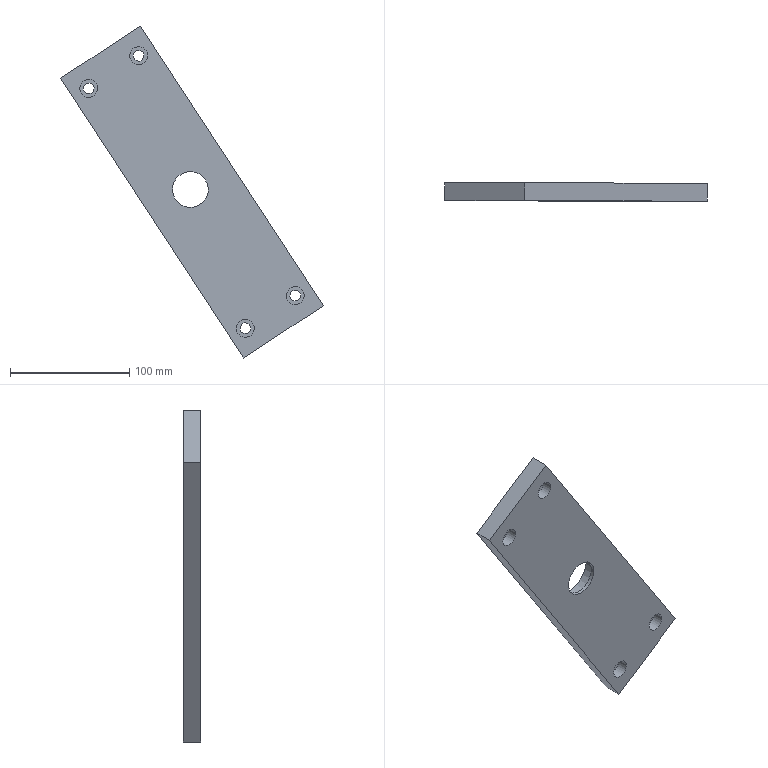Component | SolidWorks | SuctionCupRotatingShaftFixingPlate-1 | 1 solid | 31 faces | box 220.12 x 15 x 278.16 mm | volume 309366 mm3 | cylinder 20 | plane 11 | commonest cylinder face diameters 15 x8 9 x8 42 x2 30 x2 | material 6061 Alloy
build123d program:
from build123d import *

# Parameters (mm, degrees)
SKETCH1_W                                            = 80
SKETCH1_H                                            = 280
BOSS_EXTRUDE1_DEPTH                                  = 15
SKETCH2_R                                            = 15
CUT_EXTRUDE1_DEPTH                                   = 147.373
HOLE_SIZE_ACCORDING_TO_THE_TYPE_OF_HEXAG_D           = 9
HOLE_SIZE_ACCORDING_TO_THE_TYPE_OF_HEXAG_CBORE_D     = 15
HOLE_SIZE_ACCORDING_TO_THE_TYPE_OF_HEXAG_CBORE_DEPTH = 9
SKETCH5_R                                            = 21
CUT_EXTRUDE2_DEPTH                                   = 12


with BuildPart() as part:
    # Sketch1 → Boss-Extrude1 (new body)
    with BuildSketch(Plane.XY):
        Rectangle(SKETCH1_W, SKETCH1_H)
    extrude(amount=BOSS_EXTRUDE1_DEPTH)

    # Sketch2 → Cut-Extrude1 (cut, through all)
    with BuildSketch(Plane.XY.offset(15)):
        with Locations((0, 2.5)):
            Circle(SKETCH2_R)
    extrude(amount=-CUT_EXTRUDE1_DEPTH, mode=Mode.SUBTRACT)

    # Hole Size according to the type of hexag (through all)
    with Locations(Plane.XY.offset(15)):
        with Locations((-25, 120), (25, 120), (25, -120), (-25, -120)):
            CounterBoreHole(HOLE_SIZE_ACCORDING_TO_THE_TYPE_OF_HEXAG_D / 2, HOLE_SIZE_ACCORDING_TO_THE_TYPE_OF_HEXAG_CBORE_D / 2, HOLE_SIZE_ACCORDING_TO_THE_TYPE_OF_HEXAG_CBORE_DEPTH)

    # Sketch5 → Cut-Extrude2 (cut)
    with BuildSketch(Plane(origin=(0, 0, 0), x_dir=(-1, 0, 0), z_dir=(0, 0, -1))):
        with Locations((0, 2.5)):
            Circle(SKETCH5_R)
    extrude(amount=-CUT_EXTRUDE2_DEPTH, mode=Mode.SUBTRACT)


solid = part.part

# Placed as in the assembly
solid = solid.moved(Location((-27.318, 319.546, 8.337), (90, 0, 33.158)))
STEP:
#1=CARTESIAN_POINT('',(-0.4372,12.108,0.8628));
#2=VERTEX_POINT('',#1);
#3=CARTESIAN_POINT('',(-1.821,12.108,-0.04158));
#4=VERTEX_POINT('',#3);
#5=CARTESIAN_POINT('',(-1.129,12.108,0.4106));
#6=DIRECTION('',(0.,1.,-0.));
#7=DIRECTION('',(-0.8372,0.,-0.5469));
#8=AXIS2_PLACEMENT_3D('',#5,#6,#7);
#9=CIRCLE('',#8,0.8268);
#10=EDGE_CURVE('',#2,#4,#9,.T.);
#11=ORIENTED_EDGE('',*,*,#10,.F.);
#12=CARTESIAN_POINT('',(-0.4372,12.581,0.8628));
#13=VERTEX_POINT('',#12);
#14=CARTESIAN_POINT('',(-0.4372,12.108,0.8628));
#15=DIRECTION('',(0.,1.,-0.));
#16=VECTOR('',#15,39.37);
#17=LINE('',#14,#16);
#18=EDGE_CURVE('',#2,#13,#17,.T.);
#19=ORIENTED_EDGE('',*,*,#18,.T.);
#20=CARTESIAN_POINT('',(-1.821,12.581,-0.04158));
#21=VERTEX_POINT('',#20);
#22=CARTESIAN_POINT('',(-1.129,12.581,0.4106));
#23=DIRECTION('',(0.,1.,-0.));
#24=DIRECTION('',(-0.8372,0.,-0.5469));
#25=AXIS2_PLACEMENT_3D('',#22,#23,#24);
#26=CIRCLE('',#25,0.8268);
#27=EDGE_CURVE('',#13,#21,#26,.T.);
#28=ORIENTED_EDGE('',*,*,#27,.T.);
#29=CARTESIAN_POINT('',(-1.821,12.108,-0.04158));
#30=DIRECTION('',(0.,1.,-0.));
#31=VECTOR('',#30,39.37);
#32=LINE('',#29,#31);
#33=EDGE_CURVE('',#4,#21,#32,.T.);
#34=ORIENTED_EDGE('',*,*,#33,.F.);
#35=EDGE_LOOP('',(#11,#19,#28,#34));
#36=FACE_OUTER_BOUND('',#35,.T.);
#37=CARTESIAN_POINT('',(-1.129,12.108,0.4106));
#38=DIRECTION('',(0.,1.,-0.));
#39=DIRECTION('',(-0.8372,0.,-0.5469));
#40=AXIS2_PLACEMENT_3D('',#37,#38,#39);
#41=CYLINDRICAL_SURFACE('',#40,0.8268);
#42=ADVANCED_FACE('',(#36),#41,.F.);
#43=CARTESIAN_POINT('',(-4.731,12.344,3.584));
#44=VERTEX_POINT('',#43);
#45=CARTESIAN_POINT('',(-4.236,12.344,3.907));
#46=VERTEX_POINT('',#45);
#47=CARTESIAN_POINT('',(-4.483,12.344,3.745));
#48=DIRECTION('',(-0.,-1.,0.));
#49=DIRECTION('',(0.8372,0.,0.5469));
#50=AXIS2_PLACEMENT_3D('',#47,#48,#49);
#51=CIRCLE('',#50,0.2953);
#52=EDGE_CURVE('',#44,#46,#51,.T.);
#53=ORIENTED_EDGE('',*,*,#52,.F.);
#54=CARTESIAN_POINT('',(-4.731,11.99,3.584));
#55=VERTEX_POINT('',#54);
#56=CARTESIAN_POINT('',(-4.731,11.99,3.584));
#57=DIRECTION('',(-0.,-1.,0.));
#58=VECTOR('',#57,39.37);
#59=LINE('',#56,#58);
#60=EDGE_CURVE('',#44,#55,#59,.T.);
#61=ORIENTED_EDGE('',*,*,#60,.T.);
#62=CARTESIAN_POINT('',(-4.236,11.99,3.907));
#63=VERTEX_POINT('',#62);
#64=CARTESIAN_POINT('',(-4.483,11.99,3.745));
#65=DIRECTION('',(-0.,-1.,0.));
#66=DIRECTION('',(0.8372,0.,0.5469));
#67=AXIS2_PLACEMENT_3D('',#64,#65,#66);
#68=CIRCLE('',#67,0.2953);
#69=EDGE_CURVE('',#55,#63,#68,.T.);
#70=ORIENTED_EDGE('',*,*,#69,.T.);
#71=CARTESIAN_POINT('',(-4.236,11.99,3.907));
#72=DIRECTION('',(-0.,-1.,0.));
#73=VECTOR('',#72,39.37);
#74=LINE('',#71,#73);
#75=EDGE_CURVE('',#46,#63,#74,.T.);
#76=ORIENTED_EDGE('',*,*,#75,.F.);
#77=EDGE_LOOP('',(#53,#61,#70,#76));
#78=FACE_OUTER_BOUND('',#77,.T.);
#79=CARTESIAN_POINT('',(-4.483,11.99,3.745));
#80=DIRECTION('',(-0.,-1.,0.));
#81=DIRECTION('',(0.8372,0.,0.5469));
#82=AXIS2_PLACEMENT_3D('',#79,#80,#81);
#83=CYLINDRICAL_SURFACE('',#82,0.2953);
#84=ADVANCED_FACE('',(#78),#83,.F.);
#85=CARTESIAN_POINT('',(-4.632,12.581,3.648));
#86=VERTEX_POINT('',#85);
#87=CARTESIAN_POINT('',(-4.335,12.581,3.842));
#88=VERTEX_POINT('',#87);
#89=CARTESIAN_POINT('',(-4.483,12.581,3.745));
#90=DIRECTION('',(-0.,-1.,0.));
#91=DIRECTION('',(0.8372,0.,0.5469));
#92=AXIS2_PLACEMENT_3D('',#89,#90,#91);
#93=CIRCLE('',#92,0.1772);
#94=EDGE_CURVE('',#86,#88,#93,.T.);
#95=ORIENTED_EDGE('',*,*,#94,.F.);
#96=CARTESIAN_POINT('',(-4.632,12.344,3.648));
#97=VERTEX_POINT('',#96);
#98=CARTESIAN_POINT('',(-4.632,11.99,3.648));
#99=DIRECTION('',(-0.,-1.,0.));
#100=VECTOR('',#99,39.37);
#101=LINE('',#98,#100);
#102=EDGE_CURVE('',#86,#97,#101,.T.);
#103=ORIENTED_EDGE('',*,*,#102,.T.);
#104=CARTESIAN_POINT('',(-4.335,12.344,3.842));
#105=VERTEX_POINT('',#104);
#106=CARTESIAN_POINT('',(-4.483,12.344,3.745));
#107=DIRECTION('',(-0.,-1.,0.));
#108=DIRECTION('',(0.8372,0.,0.5469));
#109=AXIS2_PLACEMENT_3D('',#106,#107,#108);
#110=CIRCLE('',#109,0.1772);
#111=EDGE_CURVE('',#97,#105,#110,.T.);
#112=ORIENTED_EDGE('',*,*,#111,.T.);
#113=CARTESIAN_POINT('',(-4.335,11.99,3.842));
#114=DIRECTION('',(-0.,-1.,0.));
#115=VECTOR('',#114,39.37);
#116=LINE('',#113,#115);
#117=EDGE_CURVE('',#88,#105,#116,.T.);
#118=ORIENTED_EDGE('',*,*,#117,.F.);
#119=EDGE_LOOP('',(#95,#103,#112,#118));
#120=FACE_OUTER_BOUND('',#119,.T.);
#121=CARTESIAN_POINT('',(-4.483,11.99,3.745));
#122=DIRECTION('',(-0.,-1.,0.));
#123=DIRECTION('',(0.8372,0.,0.5469));
#124=AXIS2_PLACEMENT_3D('',#121,#122,#123);
#125=CYLINDRICAL_SURFACE('',#124,0.1772);
#126=ADVANCED_FACE('',(#120),#125,.F.);
#127=CARTESIAN_POINT('',(-3.083,12.344,4.66));
#128=VERTEX_POINT('',#127);
#129=CARTESIAN_POINT('',(-2.588,12.344,4.983));
#130=VERTEX_POINT('',#129);
#131=CARTESIAN_POINT('',(-2.835,12.344,4.822));
#132=DIRECTION('',(-0.,-1.,0.));
#133=DIRECTION('',(0.8372,0.,0.5469));
#134=AXIS2_PLACEMENT_3D('',#131,#132,#133);
#135=CIRCLE('',#134,0.2953);
#136=EDGE_CURVE('',#128,#130,#135,.T.);
#137=ORIENTED_EDGE('',*,*,#136,.F.);
#138=CARTESIAN_POINT('',(-3.083,11.99,4.66));
#139=VERTEX_POINT('',#138);
#140=CARTESIAN_POINT('',(-3.083,11.99,4.66));
#141=DIRECTION('',(-0.,-1.,0.));
#142=VECTOR('',#141,39.37);
#143=LINE('',#140,#142);
#144=EDGE_CURVE('',#128,#139,#143,.T.);
#145=ORIENTED_EDGE('',*,*,#144,.T.);
#146=CARTESIAN_POINT('',(-2.588,11.99,4.983));
#147=VERTEX_POINT('',#146);
#148=CARTESIAN_POINT('',(-2.835,11.99,4.822));
#149=DIRECTION('',(-0.,-1.,0.));
#150=DIRECTION('',(0.8372,0.,0.5469));
#151=AXIS2_PLACEMENT_3D('',#148,#149,#150);
#152=CIRCLE('',#151,0.2953);
#153=EDGE_CURVE('',#139,#147,#152,.T.);
#154=ORIENTED_EDGE('',*,*,#153,.T.);
#155=CARTESIAN_POINT('',(-2.588,11.99,4.983));
#156=DIRECTION('',(-0.,-1.,0.));
#157=VECTOR('',#156,39.37);
#158=LINE('',#155,#157);
#159=EDGE_CURVE('',#130,#147,#158,.T.);
#160=ORIENTED_EDGE('',*,*,#159,.F.);
#161=EDGE_LOOP('',(#137,#145,#154,#160));
#162=FACE_OUTER_BOUND('',#161,.T.);
#163=CARTESIAN_POINT('',(-2.835,11.99,4.822));
#164=DIRECTION('',(-0.,-1.,0.));
#165=DIRECTION('',(0.8372,0.,0.5469));
#166=AXIS2_PLACEMENT_3D('',#163,#164,#165);
#167=CYLINDRICAL_SURFACE('',#166,0.2953);
#168=ADVANCED_FACE('',(#162),#167,.F.);
#169=CARTESIAN_POINT('',(-2.984,12.581,4.725));
#170=VERTEX_POINT('',#169);
#171=CARTESIAN_POINT('',(-2.687,12.581,4.919));
#172=VERTEX_POINT('',#171);
#173=CARTESIAN_POINT('',(-2.835,12.581,4.822));
#174=DIRECTION('',(-0.,-1.,0.));
#175=DIRECTION('',(0.8372,0.,0.5469));
#176=AXIS2_PLACEMENT_3D('',#173,#174,#175);
#177=CIRCLE('',#176,0.1772);
#178=EDGE_CURVE('',#170,#172,#177,.T.);
#179=ORIENTED_EDGE('',*,*,#178,.F.);
#180=CARTESIAN_POINT('',(-2.984,12.344,4.725));
#181=VERTEX_POINT('',#180);
#182=CARTESIAN_POINT('',(-2.984,11.99,4.725));
#183=DIRECTION('',(-0.,-1.,0.));
#184=VECTOR('',#183,39.37);
#185=LINE('',#182,#184);
#186=EDGE_CURVE('',#170,#181,#185,.T.);
#187=ORIENTED_EDGE('',*,*,#186,.T.);
#188=CARTESIAN_POINT('',(-2.687,12.344,4.919));
#189=VERTEX_POINT('',#188);
#190=CARTESIAN_POINT('',(-2.835,12.344,4.822));
#191=DIRECTION('',(-0.,-1.,0.));
#192=DIRECTION('',(0.8372,0.,0.5469));
#193=AXIS2_PLACEMENT_3D('',#190,#191,#192);
#194=CIRCLE('',#193,0.1772);
#195=EDGE_CURVE('',#181,#189,#194,.T.);
#196=ORIENTED_EDGE('',*,*,#195,.T.);
#197=CARTESIAN_POINT('',(-2.687,11.99,4.919));
#198=DIRECTION('',(-0.,-1.,0.));
#199=VECTOR('',#198,39.37);
#200=LINE('',#197,#199);
#201=EDGE_CURVE('',#172,#189,#200,.T.);
#202=ORIENTED_EDGE('',*,*,#201,.F.);
#203=EDGE_LOOP('',(#179,#187,#196,#202));
#204=FACE_OUTER_BOUND('',#203,.T.);
#205=CARTESIAN_POINT('',(-2.835,11.99,4.822));
#206=DIRECTION('',(-0.,-1.,0.));
#207=DIRECTION('',(0.8372,0.,0.5469));
#208=AXIS2_PLACEMENT_3D('',#205,#206,#207);
#209=CYLINDRICAL_SURFACE('',#208,0.1772);
#210=ADVANCED_FACE('',(#204),#209,.F.);
#211=CARTESIAN_POINT('',(2.085,12.344,-3.25));
#212=VERTEX_POINT('',#211);
#213=CARTESIAN_POINT('',(2.58,12.344,-2.927));
#214=VERTEX_POINT('',#213);
#215=CARTESIAN_POINT('',(2.332,12.344,-3.089));
#216=DIRECTION('',(-0.,-1.,0.));
#217=DIRECTION('',(0.8372,0.,0.5469));
#218=AXIS2_PLACEMENT_3D('',#215,#216,#217);
#219=CIRCLE('',#218,0.2953);
#220=EDGE_CURVE('',#212,#214,#219,.T.);
#221=ORIENTED_EDGE('',*,*,#220,.F.);
#222=CARTESIAN_POINT('',(2.085,11.99,-3.25));
#223=VERTEX_POINT('',#222);
#224=CARTESIAN_POINT('',(2.085,11.99,-3.25));
#225=DIRECTION('',(-0.,-1.,0.));
#226=VECTOR('',#225,39.37);
#227=LINE('',#224,#226);
#228=EDGE_CURVE('',#212,#223,#227,.T.);
#229=ORIENTED_EDGE('',*,*,#228,.T.);
#230=CARTESIAN_POINT('',(2.58,11.99,-2.927));
#231=VERTEX_POINT('',#230);
#232=CARTESIAN_POINT('',(2.332,11.99,-3.089));
#233=DIRECTION('',(-0.,-1.,0.));
#234=DIRECTION('',(0.8372,0.,0.5469));
#235=AXIS2_PLACEMENT_3D('',#232,#233,#234);
#236=CIRCLE('',#235,0.2953);
#237=EDGE_CURVE('',#223,#231,#236,.T.);
#238=ORIENTED_EDGE('',*,*,#237,.T.);
#239=CARTESIAN_POINT('',(2.58,11.99,-2.927));
#240=DIRECTION('',(-0.,-1.,0.));
#241=VECTOR('',#240,39.37);
#242=LINE('',#239,#241);
#243=EDGE_CURVE('',#214,#231,#242,.T.);
#244=ORIENTED_EDGE('',*,*,#243,.F.);
#245=EDGE_LOOP('',(#221,#229,#238,#244));
#246=FACE_OUTER_BOUND('',#245,.T.);
#247=CARTESIAN_POINT('',(2.332,11.99,-3.089));
#248=DIRECTION('',(-0.,-1.,0.));
#249=DIRECTION('',(0.8372,0.,0.5469));
#250=AXIS2_PLACEMENT_3D('',#247,#248,#249);
#251=CYLINDRICAL_SURFACE('',#250,0.2953);
#252=ADVANCED_FACE('',(#246),#251,.F.);
#253=CARTESIAN_POINT('',(2.184,12.581,-3.185));
#254=VERTEX_POINT('',#253);
#255=CARTESIAN_POINT('',(2.481,12.581,-2.992));
#256=VERTEX_POINT('',#255);
#257=CARTESIAN_POINT('',(2.332,12.581,-3.089));
#258=DIRECTION('',(-0.,-1.,0.));
#259=DIRECTION('',(0.8372,0.,0.5469));
#260=AXIS2_PLACEMENT_3D('',#257,#258,#259);
#261=CIRCLE('',#260,0.1772);
#262=EDGE_CURVE('',#254,#256,#261,.T.);
#263=ORIENTED_EDGE('',*,*,#262,.F.);
#264=CARTESIAN_POINT('',(2.184,12.344,-3.185));
#265=VERTEX_POINT('',#264);
#266=CARTESIAN_POINT('',(2.184,11.99,-3.185));
#267=DIRECTION('',(-0.,-1.,0.));
#268=VECTOR('',#267,39.37);
#269=LINE('',#266,#268);
#270=EDGE_CURVE('',#254,#265,#269,.T.);
#271=ORIENTED_EDGE('',*,*,#270,.T.);
#272=CARTESIAN_POINT('',(2.481,12.344,-2.992));
#273=VERTEX_POINT('',#272);
#274=CARTESIAN_POINT('',(2.332,12.344,-3.089));
#275=DIRECTION('',(-0.,-1.,0.));
#276=DIRECTION('',(0.8372,0.,0.5469));
#277=AXIS2_PLACEMENT_3D('',#274,#275,#276);
#278=CIRCLE('',#277,0.1772);
#279=EDGE_CURVE('',#265,#273,#278,.T.);
#280=ORIENTED_EDGE('',*,*,#279,.T.);
#281=CARTESIAN_POINT('',(2.481,11.99,-2.992));
#282=DIRECTION('',(-0.,-1.,0.));
#283=VECTOR('',#282,39.37);
#284=LINE('',#281,#283);
#285=EDGE_CURVE('',#256,#273,#284,.T.);
#286=ORIENTED_EDGE('',*,*,#285,.F.);
#287=EDGE_LOOP('',(#263,#271,#280,#286));
#288=FACE_OUTER_BOUND('',#287,.T.);
#289=CARTESIAN_POINT('',(2.332,11.99,-3.089));
#290=DIRECTION('',(-0.,-1.,0.));
#291=DIRECTION('',(0.8372,0.,0.5469));
#292=AXIS2_PLACEMENT_3D('',#289,#290,#291);
#293=CYLINDRICAL_SURFACE('',#292,0.1772);
#294=ADVANCED_FACE('',(#288),#293,.F.);
#295=CARTESIAN_POINT('',(0.4373,12.344,-4.327));
#296=VERTEX_POINT('',#295);
#297=CARTESIAN_POINT('',(0.9317,12.344,-4.004));
#298=VERTEX_POINT('',#297);
#299=CARTESIAN_POINT('',(0.6845,12.344,-4.165));
#300=DIRECTION('',(-0.,-1.,0.));
#301=DIRECTION('',(0.8372,0.,0.5469));
#302=AXIS2_PLACEMENT_3D('',#299,#300,#301);
#303=CIRCLE('',#302,0.2953);
#304=EDGE_CURVE('',#296,#298,#303,.T.);
#305=ORIENTED_EDGE('',*,*,#304,.F.);
#306=CARTESIAN_POINT('',(0.4373,11.99,-4.327));
#307=VERTEX_POINT('',#306);
#308=CARTESIAN_POINT('',(0.4373,11.99,-4.327));
#309=DIRECTION('',(-0.,-1.,0.));
#310=VECTOR('',#309,39.37);
#311=LINE('',#308,#310);
#312=EDGE_CURVE('',#296,#307,#311,.T.);
#313=ORIENTED_EDGE('',*,*,#312,.T.);
#314=CARTESIAN_POINT('',(0.9317,11.99,-4.004));
#315=VERTEX_POINT('',#314);
#316=CARTESIAN_POINT('',(0.6845,11.99,-4.165));
#317=DIRECTION('',(-0.,-1.,0.));
#318=DIRECTION('',(0.8372,0.,0.5469));
#319=AXIS2_PLACEMENT_3D('',#316,#317,#318);
#320=CIRCLE('',#319,0.2953);
#321=EDGE_CURVE('',#307,#315,#320,.T.);
#322=ORIENTED_EDGE('',*,*,#321,.T.);
#323=CARTESIAN_POINT('',(0.9317,11.99,-4.004));
#324=DIRECTION('',(-0.,-1.,0.));
#325=VECTOR('',#324,39.37);
#326=LINE('',#323,#325);
#327=EDGE_CURVE('',#298,#315,#326,.T.);
#328=ORIENTED_EDGE('',*,*,#327,.F.);
#329=EDGE_LOOP('',(#305,#313,#322,#328));
#330=FACE_OUTER_BOUND('',#329,.T.);
#331=CARTESIAN_POINT('',(0.6845,11.99,-4.165));
#332=DIRECTION('',(-0.,-1.,0.));
#333=DIRECTION('',(0.8372,0.,0.5469));
#334=AXIS2_PLACEMENT_3D('',#331,#332,#333);
#335=CYLINDRICAL_SURFACE('',#334,0.2953);
#336=ADVANCED_FACE('',(#330),#335,.F.);
#337=CARTESIAN_POINT('',(0.5362,12.581,-4.262));
#338=VERTEX_POINT('',#337);
#339=CARTESIAN_POINT('',(0.8328,12.581,-4.068));
#340=VERTEX_POINT('',#339);
#341=CARTESIAN_POINT('',(0.6845,12.581,-4.165));
#342=DIRECTION('',(-0.,-1.,0.));
#343=DIRECTION('',(0.8372,0.,0.5469));
#344=AXIS2_PLACEMENT_3D('',#341,#342,#343);
#345=CIRCLE('',#344,0.1772);
#346=EDGE_CURVE('',#338,#340,#345,.T.);
#347=ORIENTED_EDGE('',*,*,#346,.F.);
#348=CARTESIAN_POINT('',(0.5362,12.344,-4.262));
#349=VERTEX_POINT('',#348);
#350=CARTESIAN_POINT('',(0.5362,11.99,-4.262));
#351=DIRECTION('',(-0.,-1.,0.));
#352=VECTOR('',#351,39.37);
#353=LINE('',#350,#352);
#354=EDGE_CURVE('',#338,#349,#353,.T.);
#355=ORIENTED_EDGE('',*,*,#354,.T.);
#356=CARTESIAN_POINT('',(0.8328,12.344,-4.068));
#357=VERTEX_POINT('',#356);
#358=CARTESIAN_POINT('',(0.6845,12.344,-4.165));
#359=DIRECTION('',(-0.,-1.,0.));
#360=DIRECTION('',(0.8372,0.,0.5469));
#361=AXIS2_PLACEMENT_3D('',#358,#359,#360);
#362=CIRCLE('',#361,0.1772);
#363=EDGE_CURVE('',#349,#357,#362,.T.);
#364=ORIENTED_EDGE('',*,*,#363,.T.);
#365=CARTESIAN_POINT('',(0.8328,11.99,-4.068));
#366=DIRECTION('',(-0.,-1.,0.));
#367=VECTOR('',#366,39.37);
#368=LINE('',#365,#367);
#369=EDGE_CURVE('',#340,#357,#368,.T.);
#370=ORIENTED_EDGE('',*,*,#369,.F.);
#371=EDGE_LOOP('',(#347,#355,#364,#370));
#372=FACE_OUTER_BOUND('',#371,.T.);
#373=CARTESIAN_POINT('',(0.6845,11.99,-4.165));
#374=DIRECTION('',(-0.,-1.,0.));
#375=DIRECTION('',(0.8372,0.,0.5469));
#376=AXIS2_PLACEMENT_3D('',#373,#374,#375);
#377=CYLINDRICAL_SURFACE('',#376,0.1772);
#378=ADVANCED_FACE('',(#372),#377,.F.);
#379=CARTESIAN_POINT('',(-1.624,12.108,0.08762));
#380=VERTEX_POINT('',#379);
#381=CARTESIAN_POINT('',(-0.6349,12.108,0.7336));
#382=VERTEX_POINT('',#381);
#383=CARTESIAN_POINT('',(-1.129,12.108,0.4106));
#384=DIRECTION('',(-0.,-1.,0.));
#385=DIRECTION('',(-0.8372,0.,-0.5469));
#386=AXIS2_PLACEMENT_3D('',#383,#384,#385);
#387=CIRCLE('',#386,0.5906);
#388=EDGE_CURVE('',#380,#382,#387,.T.);
#389=ORIENTED_EDGE('',*,*,#388,.F.);
#390=CARTESIAN_POINT('',(-1.624,11.99,0.08762));
#391=VERTEX_POINT('',#390);
#392=CARTESIAN_POINT('',(-1.624,12.581,0.08762));
#393=DIRECTION('',(-0.,-1.,0.));
#394=VECTOR('',#393,39.37);
#395=LINE('',#392,#394);
#396=EDGE_CURVE('',#380,#391,#395,.T.);
#397=ORIENTED_EDGE('',*,*,#396,.T.);
#398=CARTESIAN_POINT('',(-0.6349,11.99,0.7336));
#399=VERTEX_POINT('',#398);
#400=CARTESIAN_POINT('',(-1.129,11.99,0.4106));
#401=DIRECTION('',(-0.,-1.,0.));
#402=DIRECTION('',(0.8372,0.,0.5469));
#403=AXIS2_PLACEMENT_3D('',#400,#401,#402);
#404=CIRCLE('',#403,0.5906);
#405=EDGE_CURVE('',#391,#399,#404,.T.);
#406=ORIENTED_EDGE('',*,*,#405,.T.);
#407=CARTESIAN_POINT('',(-0.6349,12.581,0.7336));
#408=DIRECTION('',(-0.,-1.,0.));
#409=VECTOR('',#408,39.37);
#410=LINE('',#407,#409);
#411=EDGE_CURVE('',#382,#399,#410,.T.);
#412=ORIENTED_EDGE('',*,*,#411,.F.);
#413=EDGE_LOOP('',(#389,#397,#406,#412));
#414=FACE_OUTER_BOUND('',#413,.T.);
#415=CARTESIAN_POINT('',(-1.129,12.581,0.4106));
#416=DIRECTION('',(-0.,-1.,0.));
#417=DIRECTION('',(0.8372,0.,0.5469));
#418=AXIS2_PLACEMENT_3D('',#415,#416,#417);
#419=CYLINDRICAL_SURFACE('',#418,0.5906);
#420=ADVANCED_FACE('',(#414),#419,.F.);
#421=ORIENTED_EDGE('',*,*,#396,.F.);
#422=CARTESIAN_POINT('',(-1.129,12.108,0.4106));
#423=DIRECTION('',(-0.,-1.,0.));
#424=DIRECTION('',(-0.8372,0.,-0.5469));
#425=AXIS2_PLACEMENT_3D('',#422,#423,#424);
#426=CIRCLE('',#425,0.5906);
#427=EDGE_CURVE('',#382,#380,#426,.T.);
#428=ORIENTED_EDGE('',*,*,#427,.F.);
#429=ORIENTED_EDGE('',*,*,#411,.T.);
#430=CARTESIAN_POINT('',(-1.129,11.99,0.4106));
#431=DIRECTION('',(-0.,-1.,0.));
#432=DIRECTION('',(0.8372,0.,0.5469));
#433=AXIS2_PLACEMENT_3D('',#430,#431,#432);
#434=CIRCLE('',#433,0.5906);
#435=EDGE_CURVE('',#399,#391,#434,.T.);
#436=ORIENTED_EDGE('',*,*,#435,.T.);
#437=EDGE_LOOP('',(#421,#428,#429,#436));
#438=FACE_OUTER_BOUND('',#437,.T.);
#439=CARTESIAN_POINT('',(-1.129,12.581,0.4106));
#440=DIRECTION('',(-0.,-1.,0.));
#441=DIRECTION('',(0.8372,0.,0.5469));
#442=AXIS2_PLACEMENT_3D('',#439,#440,#441);
#443=CYLINDRICAL_SURFACE('',#442,0.5906);
#444=ADVANCED_FACE('',(#438),#443,.F.);
#445=CARTESIAN_POINT('',(3.258,12.581,-3.425));
#446=VERTEX_POINT('',#445);
#447=CARTESIAN_POINT('',(-2.772,12.581,5.804));
#448=VERTEX_POINT('',#447);
#449=CARTESIAN_POINT('',(3.258,12.581,-3.425));
#450=DIRECTION('',(-0.5469,0.,0.8372));
#451=VECTOR('',#450,39.37);
#452=LINE('',#449,#451);
#453=EDGE_CURVE('',#446,#448,#452,.T.);
#454=ORIENTED_EDGE('',*,*,#453,.T.);
#455=CARTESIAN_POINT('',(-2.772,11.99,5.804));
#456=VERTEX_POINT('',#455);
#457=CARTESIAN_POINT('',(-2.772,11.99,5.804));
#458=DIRECTION('',(0.,1.,-0.));
#459=VECTOR('',#458,39.37);
#460=LINE('',#457,#459);
#461=EDGE_CURVE('',#456,#448,#460,.T.);
#462=ORIENTED_EDGE('',*,*,#461,.F.);
#463=CARTESIAN_POINT('',(3.258,11.99,-3.425));
#464=VERTEX_POINT('',#463);
#465=CARTESIAN_POINT('',(3.258,11.99,-3.425));
#466=DIRECTION('',(-0.5469,0.,0.8372));
#467=VECTOR('',#466,39.37);
#468=LINE('',#465,#467);
#469=EDGE_CURVE('',#464,#456,#468,.T.);
#470=ORIENTED_EDGE('',*,*,#469,.F.);
#471=CARTESIAN_POINT('',(3.258,11.99,-3.425));
#472=DIRECTION('',(0.,1.,-0.));
#473=VECTOR('',#472,39.37);
#474=LINE('',#471,#473);
#475=EDGE_CURVE('',#464,#446,#474,.T.);
#476=ORIENTED_EDGE('',*,*,#475,.T.);
#477=EDGE_LOOP('',(#454,#462,#470,#476));
#478=FACE_OUTER_BOUND('',#477,.T.);
#479=CARTESIAN_POINT('',(3.258,11.99,-3.425));
#480=DIRECTION('',(-0.8372,-0.,-0.5469));
#481=DIRECTION('',(-0.,-1.,0.));
#482=AXIS2_PLACEMENT_3D('',#479,#480,#481);
#483=PLANE('',#482);
#484=ADVANCED_FACE('',(#478),#483,.F.);
#485=CARTESIAN_POINT('',(-5.409,12.581,4.081));
#486=VERTEX_POINT('',#485);
#487=CARTESIAN_POINT('',(-5.409,12.581,4.081));
#488=DIRECTION('',(-0.8372,-0.,-0.5469));
#489=VECTOR('',#488,39.37);
#490=LINE('',#487,#489);
#491=EDGE_CURVE('',#448,#486,#490,.T.);
#492=ORIENTED_EDGE('',*,*,#491,.T.);
#493=CARTESIAN_POINT('',(-5.409,11.99,4.081));
#494=VERTEX_POINT('',#493);
#495=CARTESIAN_POINT('',(-5.409,11.99,4.081));
#496=DIRECTION('',(0.,1.,-0.));
#497=VECTOR('',#496,39.37);
#498=LINE('',#495,#497);
#499=EDGE_CURVE('',#494,#486,#498,.T.);
#500=ORIENTED_EDGE('',*,*,#499,.F.);
#501=CARTESIAN_POINT('',(-5.409,11.99,4.081));
#502=DIRECTION('',(-0.8372,-0.,-0.5469));
#503=VECTOR('',#502,39.37);
#504=LINE('',#501,#503);
#505=EDGE_CURVE('',#456,#494,#504,.T.);
#506=ORIENTED_EDGE('',*,*,#505,.F.);
#507=ORIENTED_EDGE('',*,*,#461,.T.);
#508=EDGE_LOOP('',(#492,#500,#506,#507));
#509=FACE_OUTER_BOUND('',#508,.T.);
#510=CARTESIAN_POINT('',(-5.409,11.99,4.081));
#511=DIRECTION('',(0.5469,-0.,-0.8372));
#512=DIRECTION('',(0.,1.,-0.));
#513=AXIS2_PLACEMENT_3D('',#510,#511,#512);
#514=PLANE('',#513);
#515=ADVANCED_FACE('',(#509),#514,.F.);
#516=CARTESIAN_POINT('',(0.6208,12.581,-5.147));
#517=VERTEX_POINT('',#516);
#518=CARTESIAN_POINT('',(0.6208,12.581,-5.147));
#519=DIRECTION('',(0.5469,-0.,-0.8372));
#520=VECTOR('',#519,39.37);
#521=LINE('',#518,#520);
#522=EDGE_CURVE('',#486,#517,#521,.T.);
#523=ORIENTED_EDGE('',*,*,#522,.T.);
#524=CARTESIAN_POINT('',(0.6208,11.99,-5.147));
#525=VERTEX_POINT('',#524);
#526=CARTESIAN_POINT('',(0.6208,11.99,-5.147));
#527=DIRECTION('',(0.,1.,-0.));
#528=VECTOR('',#527,39.37);
#529=LINE('',#526,#528);
#530=EDGE_CURVE('',#525,#517,#529,.T.);
#531=ORIENTED_EDGE('',*,*,#530,.F.);
#532=CARTESIAN_POINT('',(0.6208,11.99,-5.147));
#533=DIRECTION('',(0.5469,-0.,-0.8372));
#534=VECTOR('',#533,39.37);
#535=LINE('',#532,#534);
#536=EDGE_CURVE('',#494,#525,#535,.T.);
#537=ORIENTED_EDGE('',*,*,#536,.F.);
#538=ORIENTED_EDGE('',*,*,#499,.T.);
#539=EDGE_LOOP('',(#523,#531,#537,#538));
#540=FACE_OUTER_BOUND('',#539,.T.);
#541=CARTESIAN_POINT('',(0.6208,11.99,-5.147));
#542=DIRECTION('',(0.8372,0.,0.5469));
#543=DIRECTION('',(0.,1.,-0.));
#544=AXIS2_PLACEMENT_3D('',#541,#542,#543);
#545=PLANE('',#544);
#546=ADVANCED_FACE('',(#540),#545,.F.);
#547=CARTESIAN_POINT('',(0.6208,12.581,-5.147));
#548=DIRECTION('',(0.8372,0.,0.5469));
#549=VECTOR('',#548,39.37);
#550=LINE('',#547,#549);
#551=EDGE_CURVE('',#517,#446,#550,.T.);
#552=ORIENTED_EDGE('',*,*,#551,.T.);
#553=ORIENTED_EDGE('',*,*,#475,.F.);
#554=CARTESIAN_POINT('',(0.6208,11.99,-5.147));
#555=DIRECTION('',(0.8372,0.,0.5469));
#556=VECTOR('',#555,39.37);
#557=LINE('',#554,#556);
#558=EDGE_CURVE('',#525,#464,#557,.T.);
#559=ORIENTED_EDGE('',*,*,#558,.F.);
#560=ORIENTED_EDGE('',*,*,#530,.T.);
#561=EDGE_LOOP('',(#552,#553,#559,#560));
#562=FACE_OUTER_BOUND('',#561,.T.);
#563=CARTESIAN_POINT('',(0.6208,11.99,-5.147));
#564=DIRECTION('',(-0.5469,0.,0.8372));
#565=DIRECTION('',(-0.,-1.,0.));
#566=AXIS2_PLACEMENT_3D('',#563,#564,#565);
#567=PLANE('',#566);
#568=ADVANCED_FACE('',(#562),#567,.F.);
#569=CARTESIAN_POINT('',(-4.483,11.99,3.745));
#570=DIRECTION('',(-0.,-1.,0.));
#571=DIRECTION('',(0.8372,0.,0.5469));
#572=AXIS2_PLACEMENT_3D('',#569,#570,#571);
#573=CIRCLE('',#572,0.2953);
#574=EDGE_CURVE('',#63,#55,#573,.T.);
#575=ORIENTED_EDGE('',*,*,#574,.F.);
#576=ORIENTED_EDGE('',*,*,#69,.F.);
#577=EDGE_LOOP('',(#575,#576));
#578=FACE_BOUND('',#577,.T.);
#579=CARTESIAN_POINT('',(-2.835,11.99,4.822));
#580=DIRECTION('',(-0.,-1.,0.));
#581=DIRECTION('',(0.8372,0.,0.5469));
#582=AXIS2_PLACEMENT_3D('',#579,#580,#581);
#583=CIRCLE('',#582,0.2953);
#584=EDGE_CURVE('',#147,#139,#583,.T.);
#585=ORIENTED_EDGE('',*,*,#584,.F.);
#586=ORIENTED_EDGE('',*,*,#153,.F.);
#587=EDGE_LOOP('',(#585,#586));
#588=FACE_BOUND('',#587,.T.);
#589=CARTESIAN_POINT('',(2.332,11.99,-3.089));
#590=DIRECTION('',(-0.,-1.,0.));
#591=DIRECTION('',(0.8372,0.,0.5469));
#592=AXIS2_PLACEMENT_3D('',#589,#590,#591);
#593=CIRCLE('',#592,0.2953);
#594=EDGE_CURVE('',#231,#223,#593,.T.);
#595=ORIENTED_EDGE('',*,*,#594,.F.);
#596=ORIENTED_EDGE('',*,*,#237,.F.);
#597=EDGE_LOOP('',(#595,#596));
#598=FACE_BOUND('',#597,.T.);
#599=CARTESIAN_POINT('',(0.6845,11.99,-4.165));
#600=DIRECTION('',(-0.,-1.,0.));
#601=DIRECTION('',(0.8372,0.,0.5469));
#602=AXIS2_PLACEMENT_3D('',#599,#600,#601);
#603=CIRCLE('',#602,0.2953);
#604=EDGE_CURVE('',#315,#307,#603,.T.);
#605=ORIENTED_EDGE('',*,*,#604,.F.);
#606=ORIENTED_EDGE('',*,*,#321,.F.);
#607=EDGE_LOOP('',(#605,#606));
#608=FACE_BOUND('',#607,.T.);
#609=ORIENTED_EDGE('',*,*,#435,.F.);
#610=ORIENTED_EDGE('',*,*,#405,.F.);
#611=EDGE_LOOP('',(#609,#610));
#612=FACE_BOUND('',#611,.T.);
#613=ORIENTED_EDGE('',*,*,#469,.T.);
#614=ORIENTED_EDGE('',*,*,#505,.T.);
#615=ORIENTED_EDGE('',*,*,#536,.T.);
#616=ORIENTED_EDGE('',*,*,#558,.T.);
#617=EDGE_LOOP('',(#613,#614,#615,#616));
#618=FACE_OUTER_BOUND('',#617,.T.);
#619=CARTESIAN_POINT('',(-1.075,11.99,0.3282));
#620=DIRECTION('',(0.,1.,-0.));
#621=DIRECTION('',(-0.8372,-0.,-0.5469));
#622=AXIS2_PLACEMENT_3D('',#619,#620,#621);
#623=PLANE('',#622);
#624=ADVANCED_FACE('',(#578,#588,#598,#608,#612,#618),#623,.F.);
#625=CARTESIAN_POINT('',(-1.129,12.581,0.4106));
#626=DIRECTION('',(0.,1.,-0.));
#627=DIRECTION('',(-0.8372,0.,-0.5469));
#628=AXIS2_PLACEMENT_3D('',#625,#626,#627);
#629=CIRCLE('',#628,0.8268);
#630=EDGE_CURVE('',#21,#13,#629,.T.);
#631=ORIENTED_EDGE('',*,*,#630,.F.);
#632=ORIENTED_EDGE('',*,*,#27,.F.);
#633=EDGE_LOOP('',(#631,#632));
#634=FACE_BOUND('',#633,.T.);
#635=CARTESIAN_POINT('',(-4.483,12.581,3.745));
#636=DIRECTION('',(-0.,-1.,0.));
#637=DIRECTION('',(0.8372,0.,0.5469));
#638=AXIS2_PLACEMENT_3D('',#635,#636,#637);
#639=CIRCLE('',#638,0.1772);
#640=EDGE_CURVE('',#88,#86,#639,.T.);
#641=ORIENTED_EDGE('',*,*,#640,.T.);
#642=ORIENTED_EDGE('',*,*,#94,.T.);
#643=EDGE_LOOP('',(#641,#642));
#644=FACE_BOUND('',#643,.T.);
#645=CARTESIAN_POINT('',(-2.835,12.581,4.822));
#646=DIRECTION('',(-0.,-1.,0.));
#647=DIRECTION('',(0.8372,0.,0.5469));
#648=AXIS2_PLACEMENT_3D('',#645,#646,#647);
#649=CIRCLE('',#648,0.1772);
#650=EDGE_CURVE('',#172,#170,#649,.T.);
#651=ORIENTED_EDGE('',*,*,#650,.T.);
#652=ORIENTED_EDGE('',*,*,#178,.T.);
#653=EDGE_LOOP('',(#651,#652));
#654=FACE_BOUND('',#653,.T.);
#655=CARTESIAN_POINT('',(2.332,12.581,-3.089));
#656=DIRECTION('',(-0.,-1.,0.));
#657=DIRECTION('',(0.8372,0.,0.5469));
#658=AXIS2_PLACEMENT_3D('',#655,#656,#657);
#659=CIRCLE('',#658,0.1772);
#660=EDGE_CURVE('',#256,#254,#659,.T.);
#661=ORIENTED_EDGE('',*,*,#660,.T.);
#662=ORIENTED_EDGE('',*,*,#262,.T.);
#663=EDGE_LOOP('',(#661,#662));
#664=FACE_BOUND('',#663,.T.);
#665=CARTESIAN_POINT('',(0.6845,12.581,-4.165));
#666=DIRECTION('',(-0.,-1.,0.));
#667=DIRECTION('',(0.8372,0.,0.5469));
#668=AXIS2_PLACEMENT_3D('',#665,#666,#667);
#669=CIRCLE('',#668,0.1772);
#670=EDGE_CURVE('',#340,#338,#669,.T.);
#671=ORIENTED_EDGE('',*,*,#670,.T.);
#672=ORIENTED_EDGE('',*,*,#346,.T.);
#673=EDGE_LOOP('',(#671,#672));
#674=FACE_BOUND('',#673,.T.);
#675=ORIENTED_EDGE('',*,*,#453,.F.);
#676=ORIENTED_EDGE('',*,*,#551,.F.);
#677=ORIENTED_EDGE('',*,*,#522,.F.);
#678=ORIENTED_EDGE('',*,*,#491,.F.);
#679=EDGE_LOOP('',(#675,#676,#677,#678));
#680=FACE_OUTER_BOUND('',#679,.T.);
#681=CARTESIAN_POINT('',(-1.075,12.581,0.3282));
#682=DIRECTION('',(0.,1.,-0.));
#683=DIRECTION('',(-0.8372,-0.,-0.5469));
#684=AXIS2_PLACEMENT_3D('',#681,#682,#683);
#685=PLANE('',#684);
#686=ADVANCED_FACE('',(#634,#644,#654,#664,#674,#680),#685,.T.);
#687=ORIENTED_EDGE('',*,*,#354,.F.);
#688=ORIENTED_EDGE('',*,*,#670,.F.);
#689=ORIENTED_EDGE('',*,*,#369,.T.);
#690=CARTESIAN_POINT('',(0.6845,12.344,-4.165));
#691=DIRECTION('',(-0.,-1.,0.));
#692=DIRECTION('',(0.8372,0.,0.5469));
#693=AXIS2_PLACEMENT_3D('',#690,#691,#692);
#694=CIRCLE('',#693,0.1772);
#695=EDGE_CURVE('',#357,#349,#694,.T.);
#696=ORIENTED_EDGE('',*,*,#695,.T.);
#697=EDGE_LOOP('',(#687,#688,#689,#696));
#698=FACE_OUTER_BOUND('',#697,.T.);
#699=CARTESIAN_POINT('',(0.6845,11.99,-4.165));
#700=DIRECTION('',(-0.,-1.,0.));
#701=DIRECTION('',(0.8372,0.,0.5469));
#702=AXIS2_PLACEMENT_3D('',#699,#700,#701);
#703=CYLINDRICAL_SURFACE('',#702,0.1772);
#704=ADVANCED_FACE('',(#698),#703,.F.);
#705=ORIENTED_EDGE('',*,*,#695,.F.);
#706=ORIENTED_EDGE('',*,*,#363,.F.);
#707=EDGE_LOOP('',(#705,#706));
#708=FACE_BOUND('',#707,.T.);
#709=CARTESIAN_POINT('',(0.6845,12.344,-4.165));
#710=DIRECTION('',(-0.,-1.,0.));
#711=DIRECTION('',(0.8372,0.,0.5469));
#712=AXIS2_PLACEMENT_3D('',#709,#710,#711);
#713=CIRCLE('',#712,0.2953);
#714=EDGE_CURVE('',#298,#296,#713,.T.);
#715=ORIENTED_EDGE('',*,*,#714,.T.);
#716=ORIENTED_EDGE('',*,*,#304,.T.);
#717=EDGE_LOOP('',(#715,#716));
#718=FACE_OUTER_BOUND('',#717,.T.);
#719=CARTESIAN_POINT('',(0.8328,12.344,-4.068));
#720=DIRECTION('',(0.,1.,-0.));
#721=DIRECTION('',(-0.8372,-0.,-0.5469));
#722=AXIS2_PLACEMENT_3D('',#719,#720,#721);
#723=PLANE('',#722);
#724=ADVANCED_FACE('',(#708,#718),#723,.F.);
#725=ORIENTED_EDGE('',*,*,#312,.F.);
#726=ORIENTED_EDGE('',*,*,#714,.F.);
#727=ORIENTED_EDGE('',*,*,#327,.T.);
#728=ORIENTED_EDGE('',*,*,#604,.T.);
#729=EDGE_LOOP('',(#725,#726,#727,#728));
#730=FACE_OUTER_BOUND('',#729,.T.);
#731=CARTESIAN_POINT('',(0.6845,11.99,-4.165));
#732=DIRECTION('',(-0.,-1.,0.));
#733=DIRECTION('',(0.8372,0.,0.5469));
#734=AXIS2_PLACEMENT_3D('',#731,#732,#733);
#735=CYLINDRICAL_SURFACE('',#734,0.2953);
#736=ADVANCED_FACE('',(#730),#735,.F.);
#737=ORIENTED_EDGE('',*,*,#270,.F.);
#738=ORIENTED_EDGE('',*,*,#660,.F.);
#739=ORIENTED_EDGE('',*,*,#285,.T.);
#740=CARTESIAN_POINT('',(2.332,12.344,-3.089));
#741=DIRECTION('',(-0.,-1.,0.));
#742=DIRECTION('',(0.8372,0.,0.5469));
#743=AXIS2_PLACEMENT_3D('',#740,#741,#742);
#744=CIRCLE('',#743,0.1772);
#745=EDGE_CURVE('',#273,#265,#744,.T.);
#746=ORIENTED_EDGE('',*,*,#745,.T.);
#747=EDGE_LOOP('',(#737,#738,#739,#746));
#748=FACE_OUTER_BOUND('',#747,.T.);
#749=CARTESIAN_POINT('',(2.332,11.99,-3.089));
#750=DIRECTION('',(-0.,-1.,0.));
#751=DIRECTION('',(0.8372,0.,0.5469));
#752=AXIS2_PLACEMENT_3D('',#749,#750,#751);
#753=CYLINDRICAL_SURFACE('',#752,0.1772);
#754=ADVANCED_FACE('',(#748),#753,.F.);
#755=ORIENTED_EDGE('',*,*,#745,.F.);
#756=ORIENTED_EDGE('',*,*,#279,.F.);
#757=EDGE_LOOP('',(#755,#756));
#758=FACE_BOUND('',#757,.T.);
#759=CARTESIAN_POINT('',(2.332,12.344,-3.089));
#760=DIRECTION('',(-0.,-1.,0.));
#761=DIRECTION('',(0.8372,0.,0.5469));
#762=AXIS2_PLACEMENT_3D('',#759,#760,#761);
#763=CIRCLE('',#762,0.2953);
#764=EDGE_CURVE('',#214,#212,#763,.T.);
#765=ORIENTED_EDGE('',*,*,#764,.T.);
#766=ORIENTED_EDGE('',*,*,#220,.T.);
#767=EDGE_LOOP('',(#765,#766));
#768=FACE_OUTER_BOUND('',#767,.T.);
#769=CARTESIAN_POINT('',(2.481,12.344,-2.992));
#770=DIRECTION('',(0.,1.,-0.));
#771=DIRECTION('',(-0.8372,-0.,-0.5469));
#772=AXIS2_PLACEMENT_3D('',#769,#770,#771);
#773=PLANE('',#772);
#774=ADVANCED_FACE('',(#758,#768),#773,.F.);
#775=ORIENTED_EDGE('',*,*,#228,.F.);
#776=ORIENTED_EDGE('',*,*,#764,.F.);
#777=ORIENTED_EDGE('',*,*,#243,.T.);
#778=ORIENTED_EDGE('',*,*,#594,.T.);
#779=EDGE_LOOP('',(#775,#776,#777,#778));
#780=FACE_OUTER_BOUND('',#779,.T.);
#781=CARTESIAN_POINT('',(2.332,11.99,-3.089));
#782=DIRECTION('',(-0.,-1.,0.));
#783=DIRECTION('',(0.8372,0.,0.5469));
#784=AXIS2_PLACEMENT_3D('',#781,#782,#783);
#785=CYLINDRICAL_SURFACE('',#784,0.2953);
#786=ADVANCED_FACE('',(#780),#785,.F.);
#787=ORIENTED_EDGE('',*,*,#186,.F.);
#788=ORIENTED_EDGE('',*,*,#650,.F.);
#789=ORIENTED_EDGE('',*,*,#201,.T.);
#790=CARTESIAN_POINT('',(-2.835,12.344,4.822));
#791=DIRECTION('',(-0.,-1.,0.));
#792=DIRECTION('',(0.8372,0.,0.5469));
#793=AXIS2_PLACEMENT_3D('',#790,#791,#792);
#794=CIRCLE('',#793,0.1772);
#795=EDGE_CURVE('',#189,#181,#794,.T.);
#796=ORIENTED_EDGE('',*,*,#795,.T.);
#797=EDGE_LOOP('',(#787,#788,#789,#796));
#798=FACE_OUTER_BOUND('',#797,.T.);
#799=CARTESIAN_POINT('',(-2.835,11.99,4.822));
#800=DIRECTION('',(-0.,-1.,0.));
#801=DIRECTION('',(0.8372,0.,0.5469));
#802=AXIS2_PLACEMENT_3D('',#799,#800,#801);
#803=CYLINDRICAL_SURFACE('',#802,0.1772);
#804=ADVANCED_FACE('',(#798),#803,.F.);
#805=ORIENTED_EDGE('',*,*,#795,.F.);
#806=ORIENTED_EDGE('',*,*,#195,.F.);
#807=EDGE_LOOP('',(#805,#806));
#808=FACE_BOUND('',#807,.T.);
#809=CARTESIAN_POINT('',(-2.835,12.344,4.822));
#810=DIRECTION('',(-0.,-1.,0.));
#811=DIRECTION('',(0.8372,0.,0.5469));
#812=AXIS2_PLACEMENT_3D('',#809,#810,#811);
#813=CIRCLE('',#812,0.2953);
#814=EDGE_CURVE('',#130,#128,#813,.T.);
#815=ORIENTED_EDGE('',*,*,#814,.T.);
#816=ORIENTED_EDGE('',*,*,#136,.T.);
#817=EDGE_LOOP('',(#815,#816));
#818=FACE_OUTER_BOUND('',#817,.T.);
#819=CARTESIAN_POINT('',(-2.687,12.344,4.919));
#820=DIRECTION('',(0.,1.,-0.));
#821=DIRECTION('',(-0.8372,-0.,-0.5469));
#822=AXIS2_PLACEMENT_3D('',#819,#820,#821);
#823=PLANE('',#822);
#824=ADVANCED_FACE('',(#808,#818),#823,.F.);
#825=ORIENTED_EDGE('',*,*,#144,.F.);
#826=ORIENTED_EDGE('',*,*,#814,.F.);
#827=ORIENTED_EDGE('',*,*,#159,.T.);
#828=ORIENTED_EDGE('',*,*,#584,.T.);
#829=EDGE_LOOP('',(#825,#826,#827,#828));
#830=FACE_OUTER_BOUND('',#829,.T.);
#831=CARTESIAN_POINT('',(-2.835,11.99,4.822));
#832=DIRECTION('',(-0.,-1.,0.));
#833=DIRECTION('',(0.8372,0.,0.5469));
#834=AXIS2_PLACEMENT_3D('',#831,#832,#833);
#835=CYLINDRICAL_SURFACE('',#834,0.2953);
#836=ADVANCED_FACE('',(#830),#835,.F.);
#837=ORIENTED_EDGE('',*,*,#102,.F.);
#838=ORIENTED_EDGE('',*,*,#640,.F.);
#839=ORIENTED_EDGE('',*,*,#117,.T.);
#840=CARTESIAN_POINT('',(-4.483,12.344,3.745));
#841=DIRECTION('',(-0.,-1.,0.));
#842=DIRECTION('',(0.8372,0.,0.5469));
#843=AXIS2_PLACEMENT_3D('',#840,#841,#842);
#844=CIRCLE('',#843,0.1772);
#845=EDGE_CURVE('',#105,#97,#844,.T.);
#846=ORIENTED_EDGE('',*,*,#845,.T.);
#847=EDGE_LOOP('',(#837,#838,#839,#846));
#848=FACE_OUTER_BOUND('',#847,.T.);
#849=CARTESIAN_POINT('',(-4.483,11.99,3.745));
#850=DIRECTION('',(-0.,-1.,0.));
#851=DIRECTION('',(0.8372,0.,0.5469));
#852=AXIS2_PLACEMENT_3D('',#849,#850,#851);
#853=CYLINDRICAL_SURFACE('',#852,0.1772);
#854=ADVANCED_FACE('',(#848),#853,.F.);
#855=ORIENTED_EDGE('',*,*,#845,.F.);
#856=ORIENTED_EDGE('',*,*,#111,.F.);
#857=EDGE_LOOP('',(#855,#856));
#858=FACE_BOUND('',#857,.T.);
#859=CARTESIAN_POINT('',(-4.483,12.344,3.745));
#860=DIRECTION('',(-0.,-1.,0.));
#861=DIRECTION('',(0.8372,0.,0.5469));
#862=AXIS2_PLACEMENT_3D('',#859,#860,#861);
#863=CIRCLE('',#862,0.2953);
#864=EDGE_CURVE('',#46,#44,#863,.T.);
#865=ORIENTED_EDGE('',*,*,#864,.T.);
#866=ORIENTED_EDGE('',*,*,#52,.T.);
#867=EDGE_LOOP('',(#865,#866));
#868=FACE_OUTER_BOUND('',#867,.T.);
#869=CARTESIAN_POINT('',(-4.335,12.344,3.842));
#870=DIRECTION('',(0.,1.,-0.));
#871=DIRECTION('',(-0.8372,-0.,-0.5469));
#872=AXIS2_PLACEMENT_3D('',#869,#870,#871);
#873=PLANE('',#872);
#874=ADVANCED_FACE('',(#858,#868),#873,.F.);
#875=ORIENTED_EDGE('',*,*,#60,.F.);
#876=ORIENTED_EDGE('',*,*,#864,.F.);
#877=ORIENTED_EDGE('',*,*,#75,.T.);
#878=ORIENTED_EDGE('',*,*,#574,.T.);
#879=EDGE_LOOP('',(#875,#876,#877,#878));
#880=FACE_OUTER_BOUND('',#879,.T.);
#881=CARTESIAN_POINT('',(-4.483,11.99,3.745));
#882=DIRECTION('',(-0.,-1.,0.));
#883=DIRECTION('',(0.8372,0.,0.5469));
#884=AXIS2_PLACEMENT_3D('',#881,#882,#883);
#885=CYLINDRICAL_SURFACE('',#884,0.2953);
#886=ADVANCED_FACE('',(#880),#885,.F.);
#887=CARTESIAN_POINT('',(-1.129,12.108,0.4106));
#888=DIRECTION('',(0.,1.,-0.));
#889=DIRECTION('',(-0.8372,0.,-0.5469));
#890=AXIS2_PLACEMENT_3D('',#887,#888,#889);
#891=CIRCLE('',#890,0.8268);
#892=EDGE_CURVE('',#4,#2,#891,.T.);
#893=ORIENTED_EDGE('',*,*,#892,.T.);
#894=ORIENTED_EDGE('',*,*,#10,.T.);
#895=EDGE_LOOP('',(#893,#894));
#896=FACE_OUTER_BOUND('',#895,.T.);
#897=ORIENTED_EDGE('',*,*,#427,.T.);
#898=ORIENTED_EDGE('',*,*,#388,.T.);
#899=EDGE_LOOP('',(#897,#898));
#900=FACE_BOUND('',#899,.T.);
#901=CARTESIAN_POINT('',(-1.129,12.108,0.4106));
#902=DIRECTION('',(0.,1.,-0.));
#903=DIRECTION('',(-0.8372,-0.,-0.5469));
#904=AXIS2_PLACEMENT_3D('',#901,#902,#903);
#905=PLANE('',#904);
#906=ADVANCED_FACE('',(#896,#900),#905,.T.);
#907=ORIENTED_EDGE('',*,*,#18,.F.);
#908=ORIENTED_EDGE('',*,*,#892,.F.);
#909=ORIENTED_EDGE('',*,*,#33,.T.);
#910=ORIENTED_EDGE('',*,*,#630,.T.);
#911=EDGE_LOOP('',(#907,#908,#909,#910));
#912=FACE_OUTER_BOUND('',#911,.T.);
#913=CARTESIAN_POINT('',(-1.129,12.108,0.4106));
#914=DIRECTION('',(0.,1.,-0.));
#915=DIRECTION('',(-0.8372,0.,-0.5469));
#916=AXIS2_PLACEMENT_3D('',#913,#914,#915);
#917=CYLINDRICAL_SURFACE('',#916,0.8268);
#918=ADVANCED_FACE('',(#912),#917,.F.);
#919=CLOSED_SHELL('',(#42,#84,#126,#168,#210,#252,#294,#336,#378,#420,#444,#484,#515,#546,#568,#624,#686,#704,#724,#736,#754,#774,#786,#804,#824,#836,#854,#874,#886,#906,#918));
#920=MANIFOLD_SOLID_BREP('',#919);
#921=CARTESIAN_POINT('',(0.,0.,0.));
#922=DIRECTION('',(0.,0.,1.));
#923=DIRECTION('',(1.,0.,0.));
#924=AXIS2_PLACEMENT_3D('',#921,#922,#923);
#925=(LENGTH_UNIT()NAMED_UNIT(*)SI_UNIT($,.METRE.));
#926=LENGTH_MEASURE_WITH_UNIT(LENGTH_MEASURE(0.0254),#925);
#927=DIMENSIONAL_EXPONENTS(1.,0.,0.,0.,0.,0.,0.);
#928=(CONVERSION_BASED_UNIT('',#926)LENGTH_UNIT()NAMED_UNIT(#927));
#929=UNCERTAINTY_MEASURE_WITH_UNIT(LENGTH_MEASURE(0.00001),#928,'','');
#930=(NAMED_UNIT(*)PLANE_ANGLE_UNIT()SI_UNIT($,.RADIAN.));
#931=(NAMED_UNIT(*)SI_UNIT($,.STERADIAN.)SOLID_ANGLE_UNIT());
#932=(GEOMETRIC_REPRESENTATION_CONTEXT(3)GLOBAL_UNCERTAINTY_ASSIGNED_CONTEXT((#929))GLOBAL_UNIT_ASSIGNED_CONTEXT((#928,#930,#931))REPRESENTATION_CONTEXT('',''));
#933=ADVANCED_BREP_SHAPE_REPRESENTATION('',(#920,#924),#932);
#934=COLOUR_RGB('',0.7922,0.8196,0.9333);
#935=FILL_AREA_STYLE_COLOUR('',#934);
#936=FILL_AREA_STYLE('',(#935));
#937=SURFACE_STYLE_FILL_AREA(#936);
#938=SURFACE_SIDE_STYLE('',(#937));
#939=SURFACE_STYLE_USAGE(.BOTH.,#938);
#940=PRESENTATION_STYLE_ASSIGNMENT((#939));
#941=STYLED_ITEM('',(#940),#920);
#942=PRESENTATION_LAYER_ASSIGNMENT('','',(#941));
#943=(LENGTH_UNIT()NAMED_UNIT(*)SI_UNIT($,.METRE.));
#944=LENGTH_MEASURE_WITH_UNIT(LENGTH_MEASURE(0.0254),#943);
#945=DIMENSIONAL_EXPONENTS(1.,0.,0.,0.,0.,0.,0.);
#946=(CONVERSION_BASED_UNIT('',#944)LENGTH_UNIT()NAMED_UNIT(#945));
#947=UNCERTAINTY_MEASURE_WITH_UNIT(LENGTH_MEASURE(0.00001),#946,'','');
#948=(NAMED_UNIT(*)PLANE_ANGLE_UNIT()SI_UNIT($,.RADIAN.));
#949=(NAMED_UNIT(*)SI_UNIT($,.STERADIAN.)SOLID_ANGLE_UNIT());
#950=(GEOMETRIC_REPRESENTATION_CONTEXT(3)GLOBAL_UNCERTAINTY_ASSIGNED_CONTEXT((#947))GLOBAL_UNIT_ASSIGNED_CONTEXT((#946,#948,#949))REPRESENTATION_CONTEXT('',''));
#951=MECHANICAL_DESIGN_GEOMETRIC_PRESENTATION_REPRESENTATION('',(#941),#950);